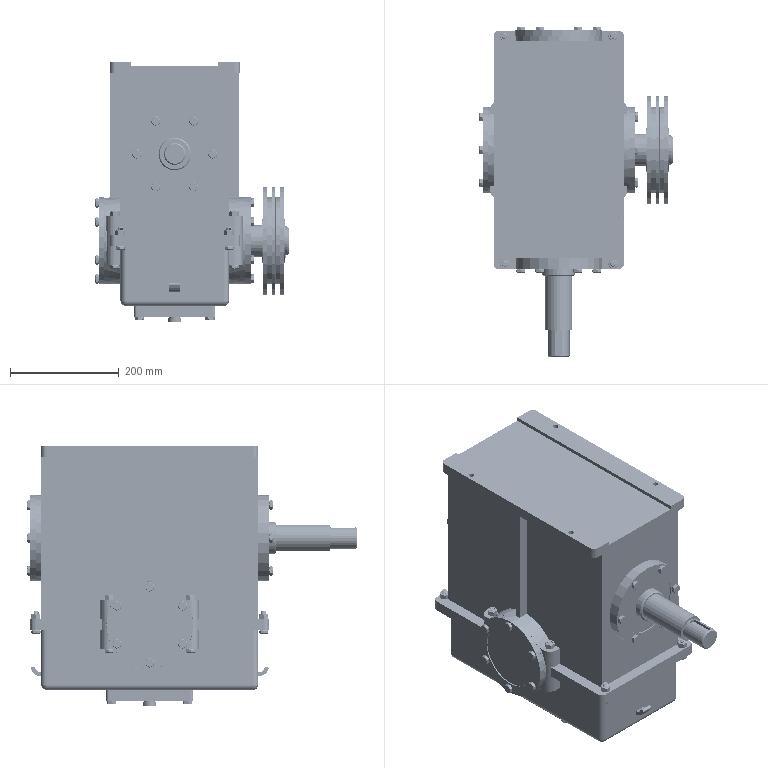Assembly | SolidWorks | mm | 56 component files | 57 solids | 2684 faces | box 356.4 x 608.4 x 480 mm | volume 15582504 mm3 | cylinder 1440 | plane 692 | cone 400 | spline 74 | torus 74 | sphere 4 | commonest cylinder face diameters 10 x1146 210 x74 120 x40 190 x36 160 x29 20 x22 60 x20 15 x8
Bill of materials:
GearboxEndCover | 2 |  | Thin flat circular ring plate with a large central through-hole and six small through-holes evenly spaced on a bolt circle; a shallow circular step or recess is visible on one face.
GearboxEndCover-NoHole | 2 |  | Thin flat solid circular disc with six small through-holes evenly spaced on a bolt circle and no central opening.
GearboxTopCover | 1 |  | Square flat plate with rounded corners and four corner through-holes. A small cylindrical pin sticks up from the center of one face, and a stepped cylindrical boss with chamfered edges sticks out from the opposite face.
hexagon nuts grade c gb | 8 |  | Hexagonal prism with a plain cylindrical through-bore along its axis and chamfered edges at both ends, giving curved arc boundaries on each flat face. It looks like a hex nut.
Key1 | 1 |  | Solid prism whose profile is an elongated rectangle with two fully rounded (semicircular) ends, extruded to a constant height.
M10-100 | 8 |  | Long hex-head bolt with a slender cylindrical shank. The far end is threaded and a long plain section sits next to the head. The tip is chamfered and the head has chamfered corners.
M10-40 | 28 |  | Short hex-head bolt with a plain shank section near the head and an external thread over the rest of its length. The head is chamfered and the tip is chamfered.
Pulley1 | 1 |  | Pulley-like disc whose rim has two circumferential V-shaped grooves. A hub is offset on one side and the bore has a keyway. One face has a recessed annular pocket around the hub.
Turbine | 1 |  | Toothed wheel with many straight-cut-looking teeth around its edge. The tooth face is concave (throated) across its width, and a cylindrical hub sticks out on both sides with a central bore. Four through-holes sit in the web, and a concentric groove or step is visible on the face.
TurbineShaft | 1 |  | Stepped solid cylindrical shaft with several diameter sections and one thin raised collar ring near one end. The ends are chamfered.
WormGearReducerLowerCasing | 1 |  | Rectangular box-shaped housing with a flat top plate and a groove along the top. A circular flanged boss on one end has a central through-hole and six bolt holes. A half-round saddle with bolting lugs sits along the bottom edge of the long side, and flanges with corner holes stick out at the base and top.
WormGearReducerUpperCasing | 1 |  | Open-top rectangular tray or box with a perimeter flange carrying bolt holes. Two semicircular cutouts are in opposite long walls and have lug features. A rectangular opening is in the inner bottom or partition area, and small hook-like protrusions are on the end walls. A raised pad is on the underside.
WormShaft | 1 |  | Stepped cylindrical shaft with a larger-diameter section in the middle carrying a helical thread-like tooth form. Several smaller stepped journal sections sit on both sides, with small grooves at the shoulders and a keyway near one end.
Mates:
1. coincident | WormGearReducerLowerCasing-1 face at (-40.429, 211.439, -165) dir (0, 0, -1) | WormGearReducerUpperCasing-1 face at (-40.429, -8.561, -165) dir (0, 0, 1)
2. coincident | WormGearReducerLowerCasing-1 edge at (79.571, 201.439, -165) dir (0, -1, 0) | WormGearReducerUpperCasing-1 edge at (79.571, 201.439, -165) dir (0, -1, 0)
3. coincident | WormGearReducerLowerCasing-1 edge at (-150.429, -228.561, -165) dir (1, 0, 0) | WormGearReducerUpperCasing-1 edge at (-150.429, -228.561, -165) dir (1, 0, 0)
4. concentric | WormGearReducerLowerCasing-1 face at (-40.429, -228.561, -5) dir (0, 1, 0) r 60 | GearboxEndCover-1 face at (-40.429, -218.561, -5) dir (0, -1, 0) r 30
5. concentric | WormGearReducerLowerCasing-1 face at (-5.429, -218.561, -65.622) dir (0, 1, 0) r 5 | GearboxEndCover-1 face at (-5.429, -218.561, -65.622) dir (0, -1, 0) r 5
6. coincident | WormGearReducerUpperCasing-1 face at (34.571, -88.561, -295) dir (0, 0, -1) | GearboxTopCover-1 face at (-40.429, -8.561, -295) dir (0, 0, 1)
7. coincident | WormGearReducerUpperCasing-1 edge at (34.571, 66.439, -295) dir (0, -1, 0) | GearboxTopCover-1 edge at (34.571, 66.439, -295) dir (0, -1, 0)
8. coincident | WormGearReducerUpperCasing-1 edge at (-110.429, 71.439, -295) dir (1, 0, 0) | GearboxTopCover-1 edge at (29.571, 71.439, -295) dir (-1, 0, 0)
9. coincident | WormGearReducerLowerCasing-1 face at (89.571, -8.561, -5) dir (1, 0, 0) | GearboxEndCover-2 face at (89.571, 143.982, -253.071) dir (-1, 0, 0)
10. concentric | WormGearReducerUpperCasing-1 face at (49.571, 52.06, -200) dir (1, 0, 0) r 5 | GearboxEndCover-2 face at (89.571, 52.06, -200) dir (1, 0, 0) r 5
11. concentric | WormGearReducerLowerCasing-1 face at (-195.429, -8.561, -165) dir (1, 0, 0) r 60 | GearboxEndCover-2 face at (89.571, -8.561, -165) dir (1, 0, 0) r 30
12. concentric | WormGearReducerLowerCasing-1 face at (-40.429, -228.561, -5) dir (0, 1, 0) r 60 | GearboxEndCover-NoHole-1 face at (-40.429, 201.439, -5) dir (0, 1, 0) r 80
13. concentric | WormGearReducerLowerCasing-1 face at (-40.429, -228.561, -5) dir (0, 1, 0) r 60 | WormShaft-1 face at (-40.429, -497.848, -5) dir (0, -1, 0) r 30
14. coincident | WormGearReducerLowerCasing-1 face at (-170.429, -8.561, -5) dir (-1, 0, 0) | GearboxEndCover-NoHole-2 face at (-170.429, 143.982, -76.929) dir (1, 0, 0)
15. concentric | WormGearReducerLowerCasing-1 face at (-170.429, -69.183, -130) dir (1, 0, 0) r 5 | GearboxEndCover-NoHole-2 face at (-170.429, -69.183, -130) dir (-1, 0, 0) r 5
16. concentric | WormGearReducerLowerCasing-1 face at (-195.429, -8.561, -165) dir (1, 0, 0) r 60 | GearboxEndCover-NoHole-2 face at (-170.429, -8.561, -165) dir (-1, 0, 0) r 80
17. coincident | WormShaft-1 face at (-70.427, 201.439, -5.377) dir (0, 1, 0) | GearboxEndCover-NoHole-1 face at (47.642, 201.439, -157.543) dir (0, -1, 0)
18. coincident | WormGearReducerLowerCasing-1 face at (-40.429, -218.561, -5) dir (0, -1, 0) | GearboxEndCover-1 face at (-216.57, -218.561, -5) dir (0, 1, 0)
19. concentric | WormGearReducerLowerCasing-1 face at (-110.429, 201.439, -5) dir (0, -1, 0) r 5 | GearboxEndCover-NoHole-1 face at (-110.429, 201.439, -5) dir (0, 1, 0) r 5
20. coincident | WormGearReducerLowerCasing-1 face at (-40.429, 201.439, -5) dir (0, 1, 0) | GearboxEndCover-NoHole-1 face at (47.642, 201.439, -157.543) dir (0, -1, 0)
21. concentric | TurbineShaft-1 face at (-170.429, -8.561, -165) dir (-1, 0, 0) r 35 | Turbine-1 face at (19.571, -8.561, -165) dir (-1, 0, 0) r 35
22. coincident | TurbineShaft-1 face at (-100.429, -48.558, -164.441) dir (1, 0, 0) | Turbine-1 face at (-100.429, -187.112, -33.955) dir (-1, 0, 0)
23. coincident | GearboxEndCover-NoHole-2 face at (-170.429, 143.982, -76.929) dir (1, 0, 0) | TurbineShaft-1 face at (-170.429, -8.561, -165) dir (-1, 0, 0)
24. concentric | GearboxEndCover-2 face at (89.571, -8.561, -165) dir (1, 0, 0) r 30 | TurbineShaft-1 face at (-170.429, -8.561, -165) dir (-1, 0, 0) r 30
25. concentric | TurbineShaft-1 face at (-170.429, -8.561, -165) dir (-1, 0, 0) r 27 | Pulley1-1 face at (119.571, -8.561, -165) dir (1, 0, 0) r 27
26. coincident | Pulley1-1 face at (113.571, -3.995, -196.067) dir (0, 0.01398, 0.9999) | Key1-1 face at (159.571, -8.995, -195.997) dir (0, -0.01398, -0.9999)
27. coincident | Pulley1-1 face at (113.571, -13.882, -187.928) dir (0, 0.9999, -0.01398) | Key1-1 face at (159.571, -13.882, -187.928) dir (0, -0.9999, 0.01398)
28. concentric | TurbineShaft-1 face at (127.571, -8.995, -195.997) dir (0, 0.01398, 0.9999) r 5 | Key1-1 face at (127.571, -8.883, -187.998) dir (0, -0.01398, -0.9999) r 5
29. coincident | TurbineShaft-1 face at (119.571, -38.558, -164.581) dir (1, 0, 0) | Pulley1-1 face at (119.571, 211.558, -168.077) dir (-1, 0, 0)
30. concentric | WormGearReducerUpperCasing-1 face at (69.571, -83.561, -210) dir (0, 0, 1) r 5 | M10-100-6 face at (69.571, -83.561, -110) dir (0, 0, -1) r 5
31. coincident | WormGearReducerUpperCasing-1 face at (-40.429, -8.561, -210) dir (0, 0, -1) | M10-100-6 face at (69.571, -83.561, -210) dir (0, 0, 1)
32. concentric | WormGearReducerUpperCasing-1 face at (59.571, 201.439, -175) dir (0, 0, 1) r 5 | M10-40-1 face at (59.571, 201.439, -140) dir (0, 0, -1) r 5
33. coincident | WormGearReducerUpperCasing-1 face at (-40.429, -8.561, -175) dir (0, 0, -1) | M10-40-1 face at (59.571, 201.439, -175) dir (0, 0, 1)
34. concentric | GearboxTopCover-1 face at (24.571, 61.439, -305) dir (0, 0, 1) r 5 | M10-100-1 face at (24.571, 61.439, -205) dir (0, 0, -1) r 5
35. coincident | GearboxTopCover-1 face at (-40.429, -8.561, -305) dir (0, 0, -1) | M10-100-1 face at (24.571, 61.439, -305) dir (0, 0, 1)
36. concentric | GearboxEndCover-NoHole-1 face at (-5.429, 201.439, -65.622) dir (0, 1, 0) r 5 | M10-40-2 face at (-5.429, 176.439, -65.622) dir (0, 1, 0) r 5
37. coincident | GearboxEndCover-NoHole-1 face at (47.642, 211.439, -157.543) dir (0, 1, 0) | M10-40-2 face at (-5.429, 211.439, -65.622) dir (0, -1, 0)
38. concentric | GearboxEndCover-2 face at (89.571, -69.183, -200) dir (1, 0, 0) r 5 | M10-40-18 face at (64.571, -69.183, -200) dir (1, 0, 0) r 5
39. coincident | GearboxEndCover-2 face at (99.571, 143.982, -253.071) dir (1, 0, 0) | M10-40-18 face at (99.571, -69.183, -200) dir (-1, 0, 0)
40. concentric | GearboxEndCover-1 face at (-110.429, -218.561, -5) dir (0, -1, 0) r 5 | M10-40-17 face at (-110.429, -193.561, -5) dir (0, -1, 0) r 5
41. coincident | GearboxEndCover-1 face at (-216.57, -228.561, -5) dir (0, -1, 0) | M10-40-17 face at (-110.429, -228.561, -5) dir (0, 1, 0)
42. concentric | GearboxEndCover-NoHole-2 face at (-170.429, -8.561, -95) dir (-1, 0, 0) r 5 | M10-40-19 face at (-145.429, -8.561, -95) dir (-1, 0, 0) r 5
43. coincident | GearboxEndCover-NoHole-2 face at (-180.429, 143.982, -76.929) dir (-1, 0, 0) | M10-40-19 face at (-180.429, -8.561, -95) dir (1, 0, 0)
44. concentric | M10-100-6 face at (69.571, -83.561, -110) dir (0, 0, -1) r 5 | hexagon nuts grade c gb-1 face at (69.571, -83.561, -120) dir (0, 0, 1) r 5
45. coincident | WormGearReducerLowerCasing-1 face at (-40.429, -8.561, -120) dir (0, 0, 1) | hexagon nuts grade c gb-1 face at (74.19, -91.561, -120) dir (0, 0, -1)
46. concentric | M10-40-1 face at (59.571, 201.439, -140) dir (0, 0, -1) r 5 | hexagon nuts grade c gb-10 face at (59.571, 201.439, -155) dir (0, 0, 1) r 5
47. coincident | WormGearReducerLowerCasing-1 face at (-40.429, 211.439, -155) dir (0, 0, 1) | hexagon nuts grade c gb-10 face at (64.19, 193.439, -155) dir (0, 0, -1)